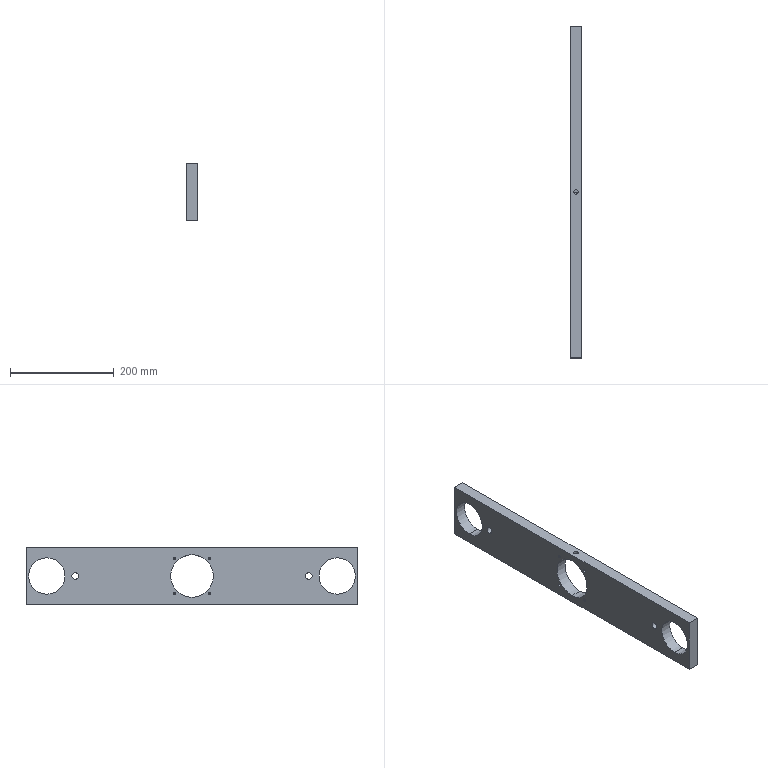Component | SolidWorks | AxisHousingBracket-2 | 1 solid | 34 faces | box 22 x 640 x 110 mm | volume 1255431 mm3 | cylinder 20 | cone 8 | plane 6 | commonest cylinder face diameters 5 x8 13 x4 70 x4 8.5 x2 82 x2
STEP:
#1=COLOUR_RGB('',0.7922,0.8196,0.9333);
#2=FILL_AREA_STYLE_COLOUR('',#1);
#3=FILL_AREA_STYLE('',(#2));
#4=SURFACE_STYLE_FILL_AREA(#3);
#5=SURFACE_SIDE_STYLE('',(#4));
#6=SURFACE_STYLE_USAGE(.BOTH.,#5);
#7=PRESENTATION_STYLE_ASSIGNMENT((#6));
#8=CARTESIAN_POINT('',(2.97,-0.1646,1.614));
#9=VERTEX_POINT('',#8);
#10=CARTESIAN_POINT('',(2.635,-0.1646,1.614));
#11=VERTEX_POINT('',#10);
#12=CARTESIAN_POINT('',(2.97,-0.1646,1.614));
#13=CARTESIAN_POINT('',(2.97,-0.1757,1.614));
#14=CARTESIAN_POINT('',(2.969,-0.1865,1.614));
#15=CARTESIAN_POINT('',(2.965,-0.2079,1.614));
#16=CARTESIAN_POINT('',(2.962,-0.2186,1.613));
#17=CARTESIAN_POINT('',(2.953,-0.2388,1.612));
#18=CARTESIAN_POINT('',(2.948,-0.2484,1.612));
#19=CARTESIAN_POINT('',(2.936,-0.2666,1.611));
#20=CARTESIAN_POINT('',(2.929,-0.2752,1.61));
#21=CARTESIAN_POINT('',(2.913,-0.2907,1.609));
#22=CARTESIAN_POINT('',(2.905,-0.2976,1.609));
#23=CARTESIAN_POINT('',(2.887,-0.3098,1.608));
#24=CARTESIAN_POINT('',(2.877,-0.315,1.607));
#25=CARTESIAN_POINT('',(2.857,-0.3233,1.606));
#26=CARTESIAN_POINT('',(2.846,-0.3266,1.606));
#27=CARTESIAN_POINT('',(2.825,-0.3309,1.606));
#28=CARTESIAN_POINT('',(2.814,-0.3319,1.605));
#29=CARTESIAN_POINT('',(2.792,-0.3319,1.605));
#30=CARTESIAN_POINT('',(2.781,-0.3308,1.606));
#31=CARTESIAN_POINT('',(2.759,-0.3266,1.606));
#32=CARTESIAN_POINT('',(2.749,-0.3234,1.606));
#33=CARTESIAN_POINT('',(2.729,-0.315,1.607));
#34=CARTESIAN_POINT('',(2.719,-0.3098,1.608));
#35=CARTESIAN_POINT('',(2.701,-0.2977,1.609));
#36=CARTESIAN_POINT('',(2.692,-0.2907,1.609));
#37=CARTESIAN_POINT('',(2.677,-0.2751,1.61));
#38=CARTESIAN_POINT('',(2.67,-0.2667,1.611));
#39=CARTESIAN_POINT('',(2.658,-0.2486,1.612));
#40=CARTESIAN_POINT('',(2.652,-0.2388,1.612));
#41=CARTESIAN_POINT('',(2.644,-0.2185,1.613));
#42=CARTESIAN_POINT('',(2.641,-0.2081,1.614));
#43=CARTESIAN_POINT('',(2.637,-0.1866,1.614));
#44=CARTESIAN_POINT('',(2.635,-0.1755,1.614));
#45=CARTESIAN_POINT('',(2.635,-0.1646,1.614));
#46=B_SPLINE_CURVE_WITH_KNOTS('',3,(#12,#13,#14,#15,#16,#17,#18,#19,#20,#21,#22,#23,#24,#25,#26,#27,#28,#29,#30,#31,#32,#33,#34,#35,#36,#37,#38,#39,#40,#41,#42,#43,#44,#45),.UNSPECIFIED.,.F.,.F.,(4,2,2,2,2,2,2,2,2,2,2,2,2,2,2,2,4),(0.,0.000831,0.001662,0.002493,0.003324,0.004155,0.004986,0.005817,0.006648,0.007479,0.00831,0.009141,0.009972,0.0108,0.01163,0.01247,0.0133),.UNSPECIFIED.);
#47=EDGE_CURVE('',#9,#11,#46,.T.);
#48=ORIENTED_EDGE('',*,*,#47,.T.);
#49=CARTESIAN_POINT('',(2.635,-0.1646,2.165));
#50=VERTEX_POINT('',#49);
#51=CARTESIAN_POINT('',(2.635,-0.1646,2.165));
#52=DIRECTION('',(0.,-0.,1.));
#53=VECTOR('',#52,39.37);
#54=LINE('',#51,#53);
#55=EDGE_CURVE('',#11,#50,#54,.T.);
#56=ORIENTED_EDGE('',*,*,#55,.T.);
#57=CARTESIAN_POINT('',(2.97,-0.1646,2.165));
#58=VERTEX_POINT('',#57);
#59=CARTESIAN_POINT('',(2.803,-0.1646,2.165));
#60=DIRECTION('',(0.,-0.,1.));
#61=DIRECTION('',(1.,0.,0.));
#62=AXIS2_PLACEMENT_3D('',#59,#60,#61);
#63=CIRCLE('',#62,0.1673);
#64=EDGE_CURVE('',#50,#58,#63,.T.);
#65=ORIENTED_EDGE('',*,*,#64,.T.);
#66=CARTESIAN_POINT('',(2.97,-0.1646,2.165));
#67=DIRECTION('',(0.,-0.,1.));
#68=VECTOR('',#67,39.37);
#69=LINE('',#66,#68);
#70=EDGE_CURVE('',#9,#58,#69,.T.);
#71=ORIENTED_EDGE('',*,*,#70,.F.);
#72=EDGE_LOOP('',(#48,#56,#65,#71));
#73=FACE_OUTER_BOUND('',#72,.T.);
#74=CARTESIAN_POINT('',(2.803,-0.1646,2.165));
#75=DIRECTION('',(0.,-0.,1.));
#76=DIRECTION('',(1.,0.,0.));
#77=AXIS2_PLACEMENT_3D('',#74,#75,#76);
#78=CYLINDRICAL_SURFACE('',#77,0.1673);
#79=ADVANCED_FACE('',(#73),#78,.F.);
#80=CARTESIAN_POINT('',(3.236,-9.023,-0.2559));
#81=VERTEX_POINT('',#80);
#82=CARTESIAN_POINT('',(3.236,-9.023,0.2559));
#83=VERTEX_POINT('',#82);
#84=CARTESIAN_POINT('',(3.236,-9.023,-0.));
#85=DIRECTION('',(-1.,0.,0.));
#86=DIRECTION('',(0.,0.,-1.));
#87=AXIS2_PLACEMENT_3D('',#84,#85,#86);
#88=CIRCLE('',#87,0.2559);
#89=EDGE_CURVE('',#81,#83,#88,.T.);
#90=ORIENTED_EDGE('',*,*,#89,.F.);
#91=CARTESIAN_POINT('',(2.37,-9.023,-0.2559));
#92=VERTEX_POINT('',#91);
#93=CARTESIAN_POINT('',(3.236,-9.023,-0.2559));
#94=DIRECTION('',(-1.,0.,0.));
#95=VECTOR('',#94,39.37);
#96=LINE('',#93,#95);
#97=EDGE_CURVE('',#81,#92,#96,.T.);
#98=ORIENTED_EDGE('',*,*,#97,.T.);
#99=CARTESIAN_POINT('',(2.37,-9.023,0.2559));
#100=VERTEX_POINT('',#99);
#101=CARTESIAN_POINT('',(2.37,-9.023,-0.));
#102=DIRECTION('',(-1.,0.,0.));
#103=DIRECTION('',(0.,0.,-1.));
#104=AXIS2_PLACEMENT_3D('',#101,#102,#103);
#105=CIRCLE('',#104,0.2559);
#106=EDGE_CURVE('',#92,#100,#105,.T.);
#107=ORIENTED_EDGE('',*,*,#106,.T.);
#108=CARTESIAN_POINT('',(3.236,-9.023,0.2559));
#109=DIRECTION('',(-1.,0.,0.));
#110=VECTOR('',#109,39.37);
#111=LINE('',#108,#110);
#112=EDGE_CURVE('',#83,#100,#111,.T.);
#113=ORIENTED_EDGE('',*,*,#112,.F.);
#114=EDGE_LOOP('',(#90,#98,#107,#113));
#115=FACE_OUTER_BOUND('',#114,.T.);
#116=CARTESIAN_POINT('',(3.236,-9.023,-0.));
#117=DIRECTION('',(-1.,0.,0.));
#118=DIRECTION('',(0.,0.,1.));
#119=AXIS2_PLACEMENT_3D('',#116,#117,#118);
#120=CYLINDRICAL_SURFACE('',#119,0.2559);
#121=ADVANCED_FACE('',(#115),#120,.F.);
#122=CARTESIAN_POINT('',(3.236,8.694,-0.2559));
#123=VERTEX_POINT('',#122);
#124=CARTESIAN_POINT('',(3.236,8.694,0.2559));
#125=VERTEX_POINT('',#124);
#126=CARTESIAN_POINT('',(3.236,8.694,0.));
#127=DIRECTION('',(-1.,0.,0.));
#128=DIRECTION('',(0.,0.,1.));
#129=AXIS2_PLACEMENT_3D('',#126,#127,#128);
#130=CIRCLE('',#129,0.2559);
#131=EDGE_CURVE('',#123,#125,#130,.T.);
#132=ORIENTED_EDGE('',*,*,#131,.F.);
#133=CARTESIAN_POINT('',(2.37,8.694,-0.2559));
#134=VERTEX_POINT('',#133);
#135=CARTESIAN_POINT('',(3.236,8.694,-0.2559));
#136=DIRECTION('',(-1.,0.,0.));
#137=VECTOR('',#136,39.37);
#138=LINE('',#135,#137);
#139=EDGE_CURVE('',#123,#134,#138,.T.);
#140=ORIENTED_EDGE('',*,*,#139,.T.);
#141=CARTESIAN_POINT('',(2.37,8.694,0.2559));
#142=VERTEX_POINT('',#141);
#143=CARTESIAN_POINT('',(2.37,8.694,0.));
#144=DIRECTION('',(-1.,0.,0.));
#145=DIRECTION('',(0.,0.,1.));
#146=AXIS2_PLACEMENT_3D('',#143,#144,#145);
#147=CIRCLE('',#146,0.2559);
#148=EDGE_CURVE('',#134,#142,#147,.T.);
#149=ORIENTED_EDGE('',*,*,#148,.T.);
#150=CARTESIAN_POINT('',(3.236,8.694,0.2559));
#151=DIRECTION('',(-1.,0.,0.));
#152=VECTOR('',#151,39.37);
#153=LINE('',#150,#152);
#154=EDGE_CURVE('',#125,#142,#153,.T.);
#155=ORIENTED_EDGE('',*,*,#154,.F.);
#156=EDGE_LOOP('',(#132,#140,#149,#155));
#157=FACE_OUTER_BOUND('',#156,.T.);
#158=CARTESIAN_POINT('',(3.236,8.694,0.));
#159=DIRECTION('',(-1.,0.,0.));
#160=DIRECTION('',(0.,0.,1.));
#161=AXIS2_PLACEMENT_3D('',#158,#159,#160);
#162=CYLINDRICAL_SURFACE('',#161,0.2559);
#163=ADVANCED_FACE('',(#157),#162,.F.);
#164=CARTESIAN_POINT('',(2.96,1.172,-1.435));
#165=VERTEX_POINT('',#164);
#166=CARTESIAN_POINT('',(2.96,1.172,-1.238));
#167=VERTEX_POINT('',#166);
#168=CARTESIAN_POINT('',(2.96,1.172,-1.336));
#169=DIRECTION('',(-1.,0.,0.));
#170=DIRECTION('',(0.,-0.,1.));
#171=AXIS2_PLACEMENT_3D('',#168,#169,#170);
#172=CIRCLE('',#171,0.09843);
#173=EDGE_CURVE('',#165,#167,#172,.T.);
#174=ORIENTED_EDGE('',*,*,#173,.F.);
#175=CARTESIAN_POINT('',(2.37,1.172,-1.435));
#176=VERTEX_POINT('',#175);
#177=CARTESIAN_POINT('',(2.37,1.172,-1.435));
#178=DIRECTION('',(-1.,0.,0.));
#179=VECTOR('',#178,39.37);
#180=LINE('',#177,#179);
#181=EDGE_CURVE('',#165,#176,#180,.T.);
#182=ORIENTED_EDGE('',*,*,#181,.T.);
#183=CARTESIAN_POINT('',(2.37,1.172,-1.238));
#184=VERTEX_POINT('',#183);
#185=CARTESIAN_POINT('',(2.37,1.172,-1.336));
#186=DIRECTION('',(-1.,0.,0.));
#187=DIRECTION('',(0.,-0.,1.));
#188=AXIS2_PLACEMENT_3D('',#185,#186,#187);
#189=CIRCLE('',#188,0.09843);
#190=EDGE_CURVE('',#176,#184,#189,.T.);
#191=ORIENTED_EDGE('',*,*,#190,.T.);
#192=CARTESIAN_POINT('',(2.37,1.172,-1.238));
#193=DIRECTION('',(-1.,0.,0.));
#194=VECTOR('',#193,39.37);
#195=LINE('',#192,#194);
#196=EDGE_CURVE('',#167,#184,#195,.T.);
#197=ORIENTED_EDGE('',*,*,#196,.F.);
#198=EDGE_LOOP('',(#174,#182,#191,#197));
#199=FACE_OUTER_BOUND('',#198,.T.);
#200=CARTESIAN_POINT('',(2.37,1.172,-1.336));
#201=DIRECTION('',(-1.,0.,0.));
#202=DIRECTION('',(0.,-0.,1.));
#203=AXIS2_PLACEMENT_3D('',#200,#201,#202);
#204=CYLINDRICAL_SURFACE('',#203,0.09843);
#205=ADVANCED_FACE('',(#199),#204,.F.);
#206=CARTESIAN_POINT('',(3.019,1.172,-1.336));
#207=VERTEX_POINT('',#206);
#208=CARTESIAN_POINT('',(2.96,1.172,-1.238));
#209=DIRECTION('',(-0.515,-0.,0.8572));
#210=VECTOR('',#209,39.37);
#211=LINE('',#208,#210);
#212=EDGE_CURVE('',#207,#167,#211,.T.);
#213=ORIENTED_EDGE('',*,*,#212,.F.);
#214=CARTESIAN_POINT('',(2.96,1.172,-1.435));
#215=DIRECTION('',(-0.515,0.,-0.8572));
#216=VECTOR('',#215,39.37);
#217=LINE('',#214,#216);
#218=EDGE_CURVE('',#207,#165,#217,.T.);
#219=ORIENTED_EDGE('',*,*,#218,.T.);
#220=ORIENTED_EDGE('',*,*,#173,.T.);
#221=EDGE_LOOP('',(#213,#219,#220));
#222=FACE_OUTER_BOUND('',#221,.T.);
#223=CARTESIAN_POINT('',(2.96,1.172,-1.336));
#224=DIRECTION('',(-1.,0.,0.));
#225=DIRECTION('',(0.,-0.,1.));
#226=AXIS2_PLACEMENT_3D('',#223,#224,#225);
#227=CONICAL_SURFACE('',#226,0.09843,1.03);
#228=ADVANCED_FACE('',(#222),#227,.F.);
#229=CARTESIAN_POINT('',(2.96,-1.501,-1.435));
#230=VERTEX_POINT('',#229);
#231=CARTESIAN_POINT('',(2.96,-1.501,-1.238));
#232=VERTEX_POINT('',#231);
#233=CARTESIAN_POINT('',(2.96,-1.501,-1.336));
#234=DIRECTION('',(-1.,0.,0.));
#235=DIRECTION('',(0.,-0.,1.));
#236=AXIS2_PLACEMENT_3D('',#233,#234,#235);
#237=CIRCLE('',#236,0.09843);
#238=EDGE_CURVE('',#230,#232,#237,.T.);
#239=ORIENTED_EDGE('',*,*,#238,.F.);
#240=CARTESIAN_POINT('',(2.37,-1.501,-1.435));
#241=VERTEX_POINT('',#240);
#242=CARTESIAN_POINT('',(2.37,-1.501,-1.435));
#243=DIRECTION('',(-1.,0.,0.));
#244=VECTOR('',#243,39.37);
#245=LINE('',#242,#244);
#246=EDGE_CURVE('',#230,#241,#245,.T.);
#247=ORIENTED_EDGE('',*,*,#246,.T.);
#248=CARTESIAN_POINT('',(2.37,-1.501,-1.238));
#249=VERTEX_POINT('',#248);
#250=CARTESIAN_POINT('',(2.37,-1.501,-1.336));
#251=DIRECTION('',(-1.,0.,0.));
#252=DIRECTION('',(0.,-0.,1.));
#253=AXIS2_PLACEMENT_3D('',#250,#251,#252);
#254=CIRCLE('',#253,0.09843);
#255=EDGE_CURVE('',#241,#249,#254,.T.);
#256=ORIENTED_EDGE('',*,*,#255,.T.);
#257=CARTESIAN_POINT('',(2.37,-1.501,-1.238));
#258=DIRECTION('',(-1.,0.,0.));
#259=VECTOR('',#258,39.37);
#260=LINE('',#257,#259);
#261=EDGE_CURVE('',#232,#249,#260,.T.);
#262=ORIENTED_EDGE('',*,*,#261,.F.);
#263=EDGE_LOOP('',(#239,#247,#256,#262));
#264=FACE_OUTER_BOUND('',#263,.T.);
#265=CARTESIAN_POINT('',(2.37,-1.501,-1.336));
#266=DIRECTION('',(-1.,0.,0.));
#267=DIRECTION('',(0.,-0.,1.));
#268=AXIS2_PLACEMENT_3D('',#265,#266,#267);
#269=CYLINDRICAL_SURFACE('',#268,0.09843);
#270=ADVANCED_FACE('',(#264),#269,.F.);
#271=CARTESIAN_POINT('',(3.019,-1.501,-1.336));
#272=VERTEX_POINT('',#271);
#273=CARTESIAN_POINT('',(2.96,-1.501,-1.238));
#274=DIRECTION('',(-0.515,-0.,0.8572));
#275=VECTOR('',#274,39.37);
#276=LINE('',#273,#275);
#277=EDGE_CURVE('',#272,#232,#276,.T.);
#278=ORIENTED_EDGE('',*,*,#277,.F.);
#279=CARTESIAN_POINT('',(2.96,-1.501,-1.435));
#280=DIRECTION('',(-0.515,0.,-0.8572));
#281=VECTOR('',#280,39.37);
#282=LINE('',#279,#281);
#283=EDGE_CURVE('',#272,#230,#282,.T.);
#284=ORIENTED_EDGE('',*,*,#283,.T.);
#285=ORIENTED_EDGE('',*,*,#238,.T.);
#286=EDGE_LOOP('',(#278,#284,#285));
#287=FACE_OUTER_BOUND('',#286,.T.);
#288=CARTESIAN_POINT('',(2.96,-1.501,-1.336));
#289=DIRECTION('',(-1.,0.,0.));
#290=DIRECTION('',(0.,-0.,1.));
#291=AXIS2_PLACEMENT_3D('',#288,#289,#290);
#292=CONICAL_SURFACE('',#291,0.09843,1.03);
#293=ADVANCED_FACE('',(#287),#292,.F.);
#294=CARTESIAN_POINT('',(2.96,-1.501,1.238));
#295=VERTEX_POINT('',#294);
#296=CARTESIAN_POINT('',(2.96,-1.501,1.435));
#297=VERTEX_POINT('',#296);
#298=CARTESIAN_POINT('',(2.96,-1.501,1.336));
#299=DIRECTION('',(-1.,0.,0.));
#300=DIRECTION('',(0.,-0.,1.));
#301=AXIS2_PLACEMENT_3D('',#298,#299,#300);
#302=CIRCLE('',#301,0.09843);
#303=EDGE_CURVE('',#295,#297,#302,.T.);
#304=ORIENTED_EDGE('',*,*,#303,.F.);
#305=CARTESIAN_POINT('',(2.37,-1.501,1.238));
#306=VERTEX_POINT('',#305);
#307=CARTESIAN_POINT('',(2.37,-1.501,1.238));
#308=DIRECTION('',(-1.,0.,0.));
#309=VECTOR('',#308,39.37);
#310=LINE('',#307,#309);
#311=EDGE_CURVE('',#295,#306,#310,.T.);
#312=ORIENTED_EDGE('',*,*,#311,.T.);
#313=CARTESIAN_POINT('',(2.37,-1.501,1.435));
#314=VERTEX_POINT('',#313);
#315=CARTESIAN_POINT('',(2.37,-1.501,1.336));
#316=DIRECTION('',(-1.,0.,0.));
#317=DIRECTION('',(0.,-0.,1.));
#318=AXIS2_PLACEMENT_3D('',#315,#316,#317);
#319=CIRCLE('',#318,0.09843);
#320=EDGE_CURVE('',#306,#314,#319,.T.);
#321=ORIENTED_EDGE('',*,*,#320,.T.);
#322=CARTESIAN_POINT('',(2.37,-1.501,1.435));
#323=DIRECTION('',(-1.,0.,0.));
#324=VECTOR('',#323,39.37);
#325=LINE('',#322,#324);
#326=EDGE_CURVE('',#297,#314,#325,.T.);
#327=ORIENTED_EDGE('',*,*,#326,.F.);
#328=EDGE_LOOP('',(#304,#312,#321,#327));
#329=FACE_OUTER_BOUND('',#328,.T.);
#330=CARTESIAN_POINT('',(2.37,-1.501,1.336));
#331=DIRECTION('',(-1.,0.,0.));
#332=DIRECTION('',(0.,-0.,1.));
#333=AXIS2_PLACEMENT_3D('',#330,#331,#332);
#334=CYLINDRICAL_SURFACE('',#333,0.09843);
#335=ADVANCED_FACE('',(#329),#334,.F.);
#336=CARTESIAN_POINT('',(3.019,-1.501,1.336));
#337=VERTEX_POINT('',#336);
#338=CARTESIAN_POINT('',(2.96,-1.501,1.435));
#339=DIRECTION('',(-0.515,-0.,0.8572));
#340=VECTOR('',#339,39.37);
#341=LINE('',#338,#340);
#342=EDGE_CURVE('',#337,#297,#341,.T.);
#343=ORIENTED_EDGE('',*,*,#342,.F.);
#344=CARTESIAN_POINT('',(2.96,-1.501,1.238));
#345=DIRECTION('',(-0.515,0.,-0.8572));
#346=VECTOR('',#345,39.37);
#347=LINE('',#344,#346);
#348=EDGE_CURVE('',#337,#295,#347,.T.);
#349=ORIENTED_EDGE('',*,*,#348,.T.);
#350=ORIENTED_EDGE('',*,*,#303,.T.);
#351=EDGE_LOOP('',(#343,#349,#350));
#352=FACE_OUTER_BOUND('',#351,.T.);
#353=CARTESIAN_POINT('',(2.96,-1.501,1.336));
#354=DIRECTION('',(-1.,0.,0.));
#355=DIRECTION('',(0.,-0.,1.));
#356=AXIS2_PLACEMENT_3D('',#353,#354,#355);
#357=CONICAL_SURFACE('',#356,0.09843,1.03);
#358=ADVANCED_FACE('',(#352),#357,.F.);
#359=CARTESIAN_POINT('',(2.96,1.172,1.238));
#360=VERTEX_POINT('',#359);
#361=CARTESIAN_POINT('',(2.96,1.172,1.435));
#362=VERTEX_POINT('',#361);
#363=CARTESIAN_POINT('',(2.96,1.172,1.336));
#364=DIRECTION('',(-1.,0.,0.));
#365=DIRECTION('',(0.,-0.,1.));
#366=AXIS2_PLACEMENT_3D('',#363,#364,#365);
#367=CIRCLE('',#366,0.09843);
#368=EDGE_CURVE('',#360,#362,#367,.T.);
#369=ORIENTED_EDGE('',*,*,#368,.F.);
#370=CARTESIAN_POINT('',(2.37,1.172,1.238));
#371=VERTEX_POINT('',#370);
#372=CARTESIAN_POINT('',(2.37,1.172,1.238));
#373=DIRECTION('',(-1.,0.,0.));
#374=VECTOR('',#373,39.37);
#375=LINE('',#372,#374);
#376=EDGE_CURVE('',#360,#371,#375,.T.);
#377=ORIENTED_EDGE('',*,*,#376,.T.);
#378=CARTESIAN_POINT('',(2.37,1.172,1.435));
#379=VERTEX_POINT('',#378);
#380=CARTESIAN_POINT('',(2.37,1.172,1.336));
#381=DIRECTION('',(-1.,0.,0.));
#382=DIRECTION('',(0.,-0.,1.));
#383=AXIS2_PLACEMENT_3D('',#380,#381,#382);
#384=CIRCLE('',#383,0.09843);
#385=EDGE_CURVE('',#371,#379,#384,.T.);
#386=ORIENTED_EDGE('',*,*,#385,.T.);
#387=CARTESIAN_POINT('',(2.37,1.172,1.435));
#388=DIRECTION('',(-1.,0.,0.));
#389=VECTOR('',#388,39.37);
#390=LINE('',#387,#389);
#391=EDGE_CURVE('',#362,#379,#390,.T.);
#392=ORIENTED_EDGE('',*,*,#391,.F.);
#393=EDGE_LOOP('',(#369,#377,#386,#392));
#394=FACE_OUTER_BOUND('',#393,.T.);
#395=CARTESIAN_POINT('',(2.37,1.172,1.336));
#396=DIRECTION('',(-1.,0.,0.));
#397=DIRECTION('',(0.,-0.,1.));
#398=AXIS2_PLACEMENT_3D('',#395,#396,#397);
#399=CYLINDRICAL_SURFACE('',#398,0.09843);
#400=ADVANCED_FACE('',(#394),#399,.F.);
#401=CARTESIAN_POINT('',(3.019,1.172,1.336));
#402=VERTEX_POINT('',#401);
#403=CARTESIAN_POINT('',(2.96,1.172,1.435));
#404=DIRECTION('',(-0.515,-0.,0.8572));
#405=VECTOR('',#404,39.37);
#406=LINE('',#403,#405);
#407=EDGE_CURVE('',#402,#362,#406,.T.);
#408=ORIENTED_EDGE('',*,*,#407,.F.);
#409=CARTESIAN_POINT('',(2.96,1.172,1.238));
#410=DIRECTION('',(-0.515,0.,-0.8572));
#411=VECTOR('',#410,39.37);
#412=LINE('',#409,#411);
#413=EDGE_CURVE('',#402,#360,#412,.T.);
#414=ORIENTED_EDGE('',*,*,#413,.T.);
#415=ORIENTED_EDGE('',*,*,#368,.T.);
#416=EDGE_LOOP('',(#408,#414,#415));
#417=FACE_OUTER_BOUND('',#416,.T.);
#418=CARTESIAN_POINT('',(2.96,1.172,1.336));
#419=DIRECTION('',(-1.,0.,0.));
#420=DIRECTION('',(0.,-0.,1.));
#421=AXIS2_PLACEMENT_3D('',#418,#419,#420);
#422=CONICAL_SURFACE('',#421,0.09843,1.03);
#423=ADVANCED_FACE('',(#417),#422,.F.);
#424=CARTESIAN_POINT('',(2.37,-11.188,-1.378));
#425=VERTEX_POINT('',#424);
#426=CARTESIAN_POINT('',(2.37,-11.188,1.378));
#427=VERTEX_POINT('',#426);
#428=CARTESIAN_POINT('',(2.37,-11.188,-0.));
#429=DIRECTION('',(-1.,0.,0.));
#430=DIRECTION('',(0.,0.,-1.));
#431=AXIS2_PLACEMENT_3D('',#428,#429,#430);
#432=CIRCLE('',#431,1.378);
#433=EDGE_CURVE('',#425,#427,#432,.T.);
#434=ORIENTED_EDGE('',*,*,#433,.T.);
#435=CARTESIAN_POINT('',(3.236,-11.188,1.378));
#436=VERTEX_POINT('',#435);
#437=CARTESIAN_POINT('',(2.37,-11.188,1.378));
#438=DIRECTION('',(1.,0.,0.));
#439=VECTOR('',#438,39.37);
#440=LINE('',#437,#439);
#441=EDGE_CURVE('',#427,#436,#440,.T.);
#442=ORIENTED_EDGE('',*,*,#441,.T.);
#443=CARTESIAN_POINT('',(3.236,-11.188,-1.378));
#444=VERTEX_POINT('',#443);
#445=CARTESIAN_POINT('',(3.236,-11.188,-0.));
#446=DIRECTION('',(-1.,0.,0.));
#447=DIRECTION('',(0.,0.,-1.));
#448=AXIS2_PLACEMENT_3D('',#445,#446,#447);
#449=CIRCLE('',#448,1.378);
#450=EDGE_CURVE('',#444,#436,#449,.T.);
#451=ORIENTED_EDGE('',*,*,#450,.F.);
#452=CARTESIAN_POINT('',(2.37,-11.188,-1.378));
#453=DIRECTION('',(1.,0.,0.));
#454=VECTOR('',#453,39.37);
#455=LINE('',#452,#454);
#456=EDGE_CURVE('',#425,#444,#455,.T.);
#457=ORIENTED_EDGE('',*,*,#456,.F.);
#458=EDGE_LOOP('',(#434,#442,#451,#457));
#459=FACE_OUTER_BOUND('',#458,.T.);
#460=CARTESIAN_POINT('',(2.37,-11.188,-0.));
#461=DIRECTION('',(1.,0.,0.));
#462=DIRECTION('',(0.,0.,-1.));
#463=AXIS2_PLACEMENT_3D('',#460,#461,#462);
#464=CYLINDRICAL_SURFACE('',#463,1.378);
#465=ADVANCED_FACE('',(#459),#464,.F.);
#466=CARTESIAN_POINT('',(2.37,10.859,-1.378));
#467=VERTEX_POINT('',#466);
#468=CARTESIAN_POINT('',(2.37,10.859,1.378));
#469=VERTEX_POINT('',#468);
#470=CARTESIAN_POINT('',(2.37,10.859,0.));
#471=DIRECTION('',(-1.,0.,0.));
#472=DIRECTION('',(0.,-0.,1.));
#473=AXIS2_PLACEMENT_3D('',#470,#471,#472);
#474=CIRCLE('',#473,1.378);
#475=EDGE_CURVE('',#467,#469,#474,.T.);
#476=ORIENTED_EDGE('',*,*,#475,.T.);
#477=CARTESIAN_POINT('',(3.236,10.859,1.378));
#478=VERTEX_POINT('',#477);
#479=CARTESIAN_POINT('',(2.37,10.859,1.378));
#480=DIRECTION('',(1.,0.,0.));
#481=VECTOR('',#480,39.37);
#482=LINE('',#479,#481);
#483=EDGE_CURVE('',#469,#478,#482,.T.);
#484=ORIENTED_EDGE('',*,*,#483,.T.);
#485=CARTESIAN_POINT('',(3.236,10.859,-1.378));
#486=VERTEX_POINT('',#485);
#487=CARTESIAN_POINT('',(3.236,10.859,0.));
#488=DIRECTION('',(-1.,0.,0.));
#489=DIRECTION('',(0.,-0.,1.));
#490=AXIS2_PLACEMENT_3D('',#487,#488,#489);
#491=CIRCLE('',#490,1.378);
#492=EDGE_CURVE('',#486,#478,#491,.T.);
#493=ORIENTED_EDGE('',*,*,#492,.F.);
#494=CARTESIAN_POINT('',(2.37,10.859,-1.378));
#495=DIRECTION('',(1.,0.,0.));
#496=VECTOR('',#495,39.37);
#497=LINE('',#494,#496);
#498=EDGE_CURVE('',#467,#486,#497,.T.);
#499=ORIENTED_EDGE('',*,*,#498,.F.);
#500=EDGE_LOOP('',(#476,#484,#493,#499));
#501=FACE_OUTER_BOUND('',#500,.T.);
#502=CARTESIAN_POINT('',(2.37,10.859,0.));
#503=DIRECTION('',(1.,0.,0.));
#504=DIRECTION('',(0.,0.,-1.));
#505=AXIS2_PLACEMENT_3D('',#502,#503,#504);
#506=CYLINDRICAL_SURFACE('',#505,1.378);
#507=ADVANCED_FACE('',(#501),#506,.F.);
#508=CARTESIAN_POINT('',(2.37,-0.1646,-1.614));
#509=VERTEX_POINT('',#508);
#510=CARTESIAN_POINT('',(2.37,-0.1646,1.614));
#511=VERTEX_POINT('',#510);
#512=CARTESIAN_POINT('',(2.37,-0.1646,0.));
#513=DIRECTION('',(-1.,0.,0.));
#514=DIRECTION('',(0.,-0.,1.));
#515=AXIS2_PLACEMENT_3D('',#512,#513,#514);
#516=CIRCLE('',#515,1.614);
#517=EDGE_CURVE('',#509,#511,#516,.T.);
#518=ORIENTED_EDGE('',*,*,#517,.T.);
#519=CARTESIAN_POINT('',(2.37,-0.1646,1.614));
#520=DIRECTION('',(1.,0.,0.));
#521=VECTOR('',#520,39.37);
#522=LINE('',#519,#521);
#523=EDGE_CURVE('',#511,#11,#522,.T.);
#524=ORIENTED_EDGE('',*,*,#523,.T.);
#525=ORIENTED_EDGE('',*,*,#47,.F.);
#526=CARTESIAN_POINT('',(3.236,-0.1646,1.614));
#527=VERTEX_POINT('',#526);
#528=CARTESIAN_POINT('',(2.37,-0.1646,1.614));
#529=DIRECTION('',(1.,0.,0.));
#530=VECTOR('',#529,39.37);
#531=LINE('',#528,#530);
#532=EDGE_CURVE('',#9,#527,#531,.T.);
#533=ORIENTED_EDGE('',*,*,#532,.T.);
#534=CARTESIAN_POINT('',(3.236,-0.1646,-1.614));
#535=VERTEX_POINT('',#534);
#536=CARTESIAN_POINT('',(3.236,-0.1646,0.));
#537=DIRECTION('',(-1.,0.,0.));
#538=DIRECTION('',(0.,-0.,1.));
#539=AXIS2_PLACEMENT_3D('',#536,#537,#538);
#540=CIRCLE('',#539,1.614);
#541=EDGE_CURVE('',#535,#527,#540,.T.);
#542=ORIENTED_EDGE('',*,*,#541,.F.);
#543=CARTESIAN_POINT('',(2.37,-0.1646,-1.614));
#544=DIRECTION('',(1.,0.,0.));
#545=VECTOR('',#544,39.37);
#546=LINE('',#543,#545);
#547=EDGE_CURVE('',#509,#535,#546,.T.);
#548=ORIENTED_EDGE('',*,*,#547,.F.);
#549=EDGE_LOOP('',(#518,#524,#525,#533,#542,#548));
#550=FACE_OUTER_BOUND('',#549,.T.);
#551=CARTESIAN_POINT('',(2.37,-0.1646,0.));
#552=DIRECTION('',(1.,0.,0.));
#553=DIRECTION('',(0.,0.,-1.));
#554=AXIS2_PLACEMENT_3D('',#551,#552,#553);
#555=CYLINDRICAL_SURFACE('',#554,1.614);
#556=ADVANCED_FACE('',(#550),#555,.F.);
#557=CARTESIAN_POINT('',(2.37,-9.023,-0.));
#558=DIRECTION('',(-1.,0.,0.));
#559=DIRECTION('',(0.,0.,-1.));
#560=AXIS2_PLACEMENT_3D('',#557,#558,#559);
#561=CIRCLE('',#560,0.2559);
#562=EDGE_CURVE('',#100,#92,#561,.T.);
#563=ORIENTED_EDGE('',*,*,#562,.F.);
#564=ORIENTED_EDGE('',*,*,#106,.F.);
#565=EDGE_LOOP('',(#563,#564));
#566=FACE_BOUND('',#565,.T.);
#567=CARTESIAN_POINT('',(2.37,8.694,0.));
#568=DIRECTION('',(-1.,0.,0.));
#569=DIRECTION('',(0.,0.,1.));
#570=AXIS2_PLACEMENT_3D('',#567,#568,#569);
#571=CIRCLE('',#570,0.2559);
#572=EDGE_CURVE('',#142,#134,#571,.T.);
#573=ORIENTED_EDGE('',*,*,#572,.F.);
#574=ORIENTED_EDGE('',*,*,#148,.F.);
#575=EDGE_LOOP('',(#573,#574));
#576=FACE_BOUND('',#575,.T.);
#577=CARTESIAN_POINT('',(2.37,1.172,-1.336));
#578=DIRECTION('',(-1.,0.,0.));
#579=DIRECTION('',(0.,-0.,1.));
#580=AXIS2_PLACEMENT_3D('',#577,#578,#579);
#581=CIRCLE('',#580,0.09843);
#582=EDGE_CURVE('',#184,#176,#581,.T.);
#583=ORIENTED_EDGE('',*,*,#582,.F.);
#584=ORIENTED_EDGE('',*,*,#190,.F.);
#585=EDGE_LOOP('',(#583,#584));
#586=FACE_BOUND('',#585,.T.);
#587=CARTESIAN_POINT('',(2.37,-1.501,-1.336));
#588=DIRECTION('',(-1.,0.,0.));
#589=DIRECTION('',(0.,-0.,1.));
#590=AXIS2_PLACEMENT_3D('',#587,#588,#589);
#591=CIRCLE('',#590,0.09843);
#592=EDGE_CURVE('',#249,#241,#591,.T.);
#593=ORIENTED_EDGE('',*,*,#592,.F.);
#594=ORIENTED_EDGE('',*,*,#255,.F.);
#595=EDGE_LOOP('',(#593,#594));
#596=FACE_BOUND('',#595,.T.);
#597=CARTESIAN_POINT('',(2.37,-1.501,1.336));
#598=DIRECTION('',(-1.,0.,0.));
#599=DIRECTION('',(0.,-0.,1.));
#600=AXIS2_PLACEMENT_3D('',#597,#598,#599);
#601=CIRCLE('',#600,0.09843);
#602=EDGE_CURVE('',#314,#306,#601,.T.);
#603=ORIENTED_EDGE('',*,*,#602,.F.);
#604=ORIENTED_EDGE('',*,*,#320,.F.);
#605=EDGE_LOOP('',(#603,#604));
#606=FACE_BOUND('',#605,.T.);
#607=CARTESIAN_POINT('',(2.37,1.172,1.336));
#608=DIRECTION('',(-1.,0.,0.));
#609=DIRECTION('',(0.,-0.,1.));
#610=AXIS2_PLACEMENT_3D('',#607,#608,#609);
#611=CIRCLE('',#610,0.09843);
#612=EDGE_CURVE('',#379,#371,#611,.T.);
#613=ORIENTED_EDGE('',*,*,#612,.F.);
#614=ORIENTED_EDGE('',*,*,#385,.F.);
#615=EDGE_LOOP('',(#613,#614));
#616=FACE_BOUND('',#615,.T.);
#617=ORIENTED_EDGE('',*,*,#475,.F.);
#618=CARTESIAN_POINT('',(2.37,10.859,0.));
#619=DIRECTION('',(-1.,0.,0.));
#620=DIRECTION('',(0.,-0.,1.));
#621=AXIS2_PLACEMENT_3D('',#618,#619,#620);
#622=CIRCLE('',#621,1.378);
#623=EDGE_CURVE('',#469,#467,#622,.T.);
#624=ORIENTED_EDGE('',*,*,#623,.F.);
#625=EDGE_LOOP('',(#617,#624));
#626=FACE_BOUND('',#625,.T.);
#627=CARTESIAN_POINT('',(2.37,-12.763,2.165));
#628=VERTEX_POINT('',#627);
#629=CARTESIAN_POINT('',(2.37,12.434,2.165));
#630=VERTEX_POINT('',#629);
#631=CARTESIAN_POINT('',(2.37,12.434,2.165));
#632=DIRECTION('',(0.,1.,0.));
#633=VECTOR('',#632,39.37);
#634=LINE('',#631,#633);
#635=EDGE_CURVE('',#628,#630,#634,.T.);
#636=ORIENTED_EDGE('',*,*,#635,.T.);
#637=CARTESIAN_POINT('',(2.37,12.434,-2.165));
#638=VERTEX_POINT('',#637);
#639=CARTESIAN_POINT('',(2.37,12.434,-2.165));
#640=DIRECTION('',(0.,0.,-1.));
#641=VECTOR('',#640,39.37);
#642=LINE('',#639,#641);
#643=EDGE_CURVE('',#630,#638,#642,.T.);
#644=ORIENTED_EDGE('',*,*,#643,.T.);
#645=CARTESIAN_POINT('',(2.37,-12.763,-2.165));
#646=VERTEX_POINT('',#645);
#647=CARTESIAN_POINT('',(2.37,12.434,-2.165));
#648=DIRECTION('',(0.,-1.,-0.));
#649=VECTOR('',#648,39.37);
#650=LINE('',#647,#649);
#651=EDGE_CURVE('',#638,#646,#650,.T.);
#652=ORIENTED_EDGE('',*,*,#651,.T.);
#653=CARTESIAN_POINT('',(2.37,-12.763,-2.165));
#654=DIRECTION('',(0.,-0.,1.));
#655=VECTOR('',#654,39.37);
#656=LINE('',#653,#655);
#657=EDGE_CURVE('',#646,#628,#656,.T.);
#658=ORIENTED_EDGE('',*,*,#657,.T.);
#659=EDGE_LOOP('',(#636,#644,#652,#658));
#660=FACE_OUTER_BOUND('',#659,.T.);
#661=ORIENTED_EDGE('',*,*,#517,.F.);
#662=CARTESIAN_POINT('',(2.37,-0.1646,0.));
#663=DIRECTION('',(-1.,0.,0.));
#664=DIRECTION('',(0.,-0.,1.));
#665=AXIS2_PLACEMENT_3D('',#662,#663,#664);
#666=CIRCLE('',#665,1.614);
#667=EDGE_CURVE('',#511,#509,#666,.T.);
#668=ORIENTED_EDGE('',*,*,#667,.F.);
#669=EDGE_LOOP('',(#661,#668));
#670=FACE_BOUND('',#669,.T.);
#671=ORIENTED_EDGE('',*,*,#433,.F.);
#672=CARTESIAN_POINT('',(2.37,-11.188,-0.));
#673=DIRECTION('',(-1.,0.,0.));
#674=DIRECTION('',(0.,0.,-1.));
#675=AXIS2_PLACEMENT_3D('',#672,#673,#674);
#676=CIRCLE('',#675,1.378);
#677=EDGE_CURVE('',#427,#425,#676,.T.);
#678=ORIENTED_EDGE('',*,*,#677,.F.);
#679=EDGE_LOOP('',(#671,#678));
#680=FACE_BOUND('',#679,.T.);
#681=CARTESIAN_POINT('',(2.37,-12.763,2.165));
#682=DIRECTION('',(-1.,0.,0.));
#683=DIRECTION('',(0.,-0.,1.));
#684=AXIS2_PLACEMENT_3D('',#681,#682,#683);
#685=PLANE('',#684);
#686=ADVANCED_FACE('',(#566,#576,#586,#596,#606,#616,#626,#660,#670,#680),#685,.T.);
#687=CARTESIAN_POINT('',(3.236,-9.023,-0.));
#688=DIRECTION('',(-1.,0.,0.));
#689=DIRECTION('',(0.,0.,-1.));
#690=AXIS2_PLACEMENT_3D('',#687,#688,#689);
#691=CIRCLE('',#690,0.2559);
#692=EDGE_CURVE('',#83,#81,#691,.T.);
#693=ORIENTED_EDGE('',*,*,#692,.T.);
#694=ORIENTED_EDGE('',*,*,#89,.T.);
#695=EDGE_LOOP('',(#693,#694));
#696=FACE_BOUND('',#695,.T.);
#697=CARTESIAN_POINT('',(3.236,8.694,0.));
#698=DIRECTION('',(-1.,0.,0.));
#699=DIRECTION('',(0.,0.,1.));
#700=AXIS2_PLACEMENT_3D('',#697,#698,#699);
#701=CIRCLE('',#700,0.2559);
#702=EDGE_CURVE('',#125,#123,#701,.T.);
#703=ORIENTED_EDGE('',*,*,#702,.T.);
#704=ORIENTED_EDGE('',*,*,#131,.T.);
#705=EDGE_LOOP('',(#703,#704));
#706=FACE_BOUND('',#705,.T.);
#707=CARTESIAN_POINT('',(3.236,-12.763,2.165));
#708=VERTEX_POINT('',#707);
#709=CARTESIAN_POINT('',(3.236,12.434,2.165));
#710=VERTEX_POINT('',#709);
#711=CARTESIAN_POINT('',(3.236,12.434,2.165));
#712=DIRECTION('',(0.,1.,0.));
#713=VECTOR('',#712,39.37);
#714=LINE('',#711,#713);
#715=EDGE_CURVE('',#708,#710,#714,.T.);
#716=ORIENTED_EDGE('',*,*,#715,.F.);
#717=CARTESIAN_POINT('',(3.236,-12.763,-2.165));
#718=VERTEX_POINT('',#717);
#719=CARTESIAN_POINT('',(3.236,-12.763,-2.165));
#720=DIRECTION('',(0.,-0.,1.));
#721=VECTOR('',#720,39.37);
#722=LINE('',#719,#721);
#723=EDGE_CURVE('',#718,#708,#722,.T.);
#724=ORIENTED_EDGE('',*,*,#723,.F.);
#725=CARTESIAN_POINT('',(3.236,12.434,-2.165));
#726=VERTEX_POINT('',#725);
#727=CARTESIAN_POINT('',(3.236,12.434,-2.165));
#728=DIRECTION('',(0.,-1.,-0.));
#729=VECTOR('',#728,39.37);
#730=LINE('',#727,#729);
#731=EDGE_CURVE('',#726,#718,#730,.T.);
#732=ORIENTED_EDGE('',*,*,#731,.F.);
#733=CARTESIAN_POINT('',(3.236,12.434,-2.165));
#734=DIRECTION('',(0.,0.,-1.));
#735=VECTOR('',#734,39.37);
#736=LINE('',#733,#735);
#737=EDGE_CURVE('',#710,#726,#736,.T.);
#738=ORIENTED_EDGE('',*,*,#737,.F.);
#739=EDGE_LOOP('',(#716,#724,#732,#738));
#740=FACE_OUTER_BOUND('',#739,.T.);
#741=ORIENTED_EDGE('',*,*,#541,.T.);
#742=CARTESIAN_POINT('',(3.236,-0.1646,0.));
#743=DIRECTION('',(-1.,0.,0.));
#744=DIRECTION('',(0.,-0.,1.));
#745=AXIS2_PLACEMENT_3D('',#742,#743,#744);
#746=CIRCLE('',#745,1.614);
#747=EDGE_CURVE('',#527,#535,#746,.T.);
#748=ORIENTED_EDGE('',*,*,#747,.T.);
#749=EDGE_LOOP('',(#741,#748));
#750=FACE_BOUND('',#749,.T.);
#751=ORIENTED_EDGE('',*,*,#492,.T.);
#752=CARTESIAN_POINT('',(3.236,10.859,0.));
#753=DIRECTION('',(-1.,0.,0.));
#754=DIRECTION('',(0.,-0.,1.));
#755=AXIS2_PLACEMENT_3D('',#752,#753,#754);
#756=CIRCLE('',#755,1.378);
#757=EDGE_CURVE('',#478,#486,#756,.T.);
#758=ORIENTED_EDGE('',*,*,#757,.T.);
#759=EDGE_LOOP('',(#751,#758));
#760=FACE_BOUND('',#759,.T.);
#761=ORIENTED_EDGE('',*,*,#450,.T.);
#762=CARTESIAN_POINT('',(3.236,-11.188,-0.));
#763=DIRECTION('',(-1.,0.,0.));
#764=DIRECTION('',(0.,0.,-1.));
#765=AXIS2_PLACEMENT_3D('',#762,#763,#764);
#766=CIRCLE('',#765,1.378);
#767=EDGE_CURVE('',#436,#444,#766,.T.);
#768=ORIENTED_EDGE('',*,*,#767,.T.);
#769=EDGE_LOOP('',(#761,#768));
#770=FACE_BOUND('',#769,.T.);
#771=CARTESIAN_POINT('',(3.236,-12.763,2.165));
#772=DIRECTION('',(-1.,0.,0.));
#773=DIRECTION('',(0.,-0.,1.));
#774=AXIS2_PLACEMENT_3D('',#771,#772,#773);
#775=PLANE('',#774);
#776=ADVANCED_FACE('',(#696,#706,#740,#750,#760,#770),#775,.F.);
#777=CARTESIAN_POINT('',(2.803,-0.1646,2.165));
#778=DIRECTION('',(0.,-0.,1.));
#779=DIRECTION('',(1.,0.,0.));
#780=AXIS2_PLACEMENT_3D('',#777,#778,#779);
#781=CIRCLE('',#780,0.1673);
#782=EDGE_CURVE('',#58,#50,#781,.T.);
#783=ORIENTED_EDGE('',*,*,#782,.F.);
#784=ORIENTED_EDGE('',*,*,#64,.F.);
#785=EDGE_LOOP('',(#783,#784));
#786=FACE_BOUND('',#785,.T.);
#787=ORIENTED_EDGE('',*,*,#715,.T.);
#788=CARTESIAN_POINT('',(2.37,12.434,2.165));
#789=DIRECTION('',(1.,0.,0.));
#790=VECTOR('',#789,39.37);
#791=LINE('',#788,#790);
#792=EDGE_CURVE('',#630,#710,#791,.T.);
#793=ORIENTED_EDGE('',*,*,#792,.F.);
#794=ORIENTED_EDGE('',*,*,#635,.F.);
#795=CARTESIAN_POINT('',(2.37,-12.763,2.165));
#796=DIRECTION('',(1.,0.,0.));
#797=VECTOR('',#796,39.37);
#798=LINE('',#795,#797);
#799=EDGE_CURVE('',#628,#708,#798,.T.);
#800=ORIENTED_EDGE('',*,*,#799,.T.);
#801=EDGE_LOOP('',(#787,#793,#794,#800));
#802=FACE_OUTER_BOUND('',#801,.T.);
#803=CARTESIAN_POINT('',(2.37,12.434,2.165));
#804=DIRECTION('',(0.,0.,-1.));
#805=DIRECTION('',(0.,-1.,-0.));
#806=AXIS2_PLACEMENT_3D('',#803,#804,#805);
#807=PLANE('',#806);
#808=ADVANCED_FACE('',(#786,#802),#807,.F.);
#809=ORIENTED_EDGE('',*,*,#737,.T.);
#810=CARTESIAN_POINT('',(2.37,12.434,-2.165));
#811=DIRECTION('',(1.,0.,0.));
#812=VECTOR('',#811,39.37);
#813=LINE('',#810,#812);
#814=EDGE_CURVE('',#638,#726,#813,.T.);
#815=ORIENTED_EDGE('',*,*,#814,.F.);
#816=ORIENTED_EDGE('',*,*,#643,.F.);
#817=ORIENTED_EDGE('',*,*,#792,.T.);
#818=EDGE_LOOP('',(#809,#815,#816,#817));
#819=FACE_OUTER_BOUND('',#818,.T.);
#820=CARTESIAN_POINT('',(2.37,12.434,-2.165));
#821=DIRECTION('',(0.,-1.,-0.));
#822=DIRECTION('',(1.,0.,0.));
#823=AXIS2_PLACEMENT_3D('',#820,#821,#822);
#824=PLANE('',#823);
#825=ADVANCED_FACE('',(#819),#824,.F.);
#826=ORIENTED_EDGE('',*,*,#731,.T.);
#827=CARTESIAN_POINT('',(2.37,-12.763,-2.165));
#828=DIRECTION('',(1.,0.,0.));
#829=VECTOR('',#828,39.37);
#830=LINE('',#827,#829);
#831=EDGE_CURVE('',#646,#718,#830,.T.);
#832=ORIENTED_EDGE('',*,*,#831,.F.);
#833=ORIENTED_EDGE('',*,*,#651,.F.);
#834=ORIENTED_EDGE('',*,*,#814,.T.);
#835=EDGE_LOOP('',(#826,#832,#833,#834));
#836=FACE_OUTER_BOUND('',#835,.T.);
#837=CARTESIAN_POINT('',(2.37,12.434,-2.165));
#838=DIRECTION('',(0.,-0.,1.));
#839=DIRECTION('',(0.,1.,0.));
#840=AXIS2_PLACEMENT_3D('',#837,#838,#839);
#841=PLANE('',#840);
#842=ADVANCED_FACE('',(#836),#841,.F.);
#843=ORIENTED_EDGE('',*,*,#723,.T.);
#844=ORIENTED_EDGE('',*,*,#799,.F.);
#845=ORIENTED_EDGE('',*,*,#657,.F.);
#846=ORIENTED_EDGE('',*,*,#831,.T.);
#847=EDGE_LOOP('',(#843,#844,#845,#846));
#848=FACE_OUTER_BOUND('',#847,.T.);
#849=CARTESIAN_POINT('',(2.37,-12.763,-2.165));
#850=DIRECTION('',(0.,1.,0.));
#851=DIRECTION('',(-1.,0.,0.));
#852=AXIS2_PLACEMENT_3D('',#849,#850,#851);
#853=PLANE('',#852);
#854=ADVANCED_FACE('',(#848),#853,.F.);
#855=ORIENTED_EDGE('',*,*,#523,.F.);
#856=ORIENTED_EDGE('',*,*,#667,.T.);
#857=ORIENTED_EDGE('',*,*,#547,.T.);
#858=ORIENTED_EDGE('',*,*,#747,.F.);
#859=ORIENTED_EDGE('',*,*,#532,.F.);
#860=CARTESIAN_POINT('',(2.635,-0.1646,1.614));
#861=CARTESIAN_POINT('',(2.635,-0.1537,1.614));
#862=CARTESIAN_POINT('',(2.637,-0.1428,1.614));
#863=CARTESIAN_POINT('',(2.641,-0.1212,1.614));
#864=CARTESIAN_POINT('',(2.644,-0.1107,1.613));
#865=CARTESIAN_POINT('',(2.652,-0.09053,1.613));
#866=CARTESIAN_POINT('',(2.658,-0.0808,1.612));
#867=CARTESIAN_POINT('',(2.67,-0.06251,1.611));
#868=CARTESIAN_POINT('',(2.677,-0.05409,1.61));
#869=CARTESIAN_POINT('',(2.692,-0.03865,1.609));
#870=CARTESIAN_POINT('',(2.701,-0.03159,1.609));
#871=CARTESIAN_POINT('',(2.719,-0.01944,1.608));
#872=CARTESIAN_POINT('',(2.728,-0.01429,1.607));
#873=CARTESIAN_POINT('',(2.749,-0.005882,1.606));
#874=CARTESIAN_POINT('',(2.759,-0.002653,1.606));
#875=CARTESIAN_POINT('',(2.781,0.001615,1.606));
#876=CARTESIAN_POINT('',(2.792,0.002708,1.605));
#877=CARTESIAN_POINT('',(2.814,0.002725,1.605));
#878=CARTESIAN_POINT('',(2.825,0.001646,1.606));
#879=CARTESIAN_POINT('',(2.846,-0.002592,1.606));
#880=CARTESIAN_POINT('',(2.857,-0.005802,1.606));
#881=CARTESIAN_POINT('',(2.877,-0.01419,1.607));
#882=CARTESIAN_POINT('',(2.887,-0.01932,1.608));
#883=CARTESIAN_POINT('',(2.905,-0.03145,1.609));
#884=CARTESIAN_POINT('',(2.913,-0.0385,1.609));
#885=CARTESIAN_POINT('',(2.929,-0.05392,1.61));
#886=CARTESIAN_POINT('',(2.936,-0.06233,1.611));
#887=CARTESIAN_POINT('',(2.948,-0.0806,1.612));
#888=CARTESIAN_POINT('',(2.953,-0.09033,1.612));
#889=CARTESIAN_POINT('',(2.961,-0.1104,1.613));
#890=CARTESIAN_POINT('',(2.965,-0.121,1.614));
#891=CARTESIAN_POINT('',(2.969,-0.1426,1.614));
#892=CARTESIAN_POINT('',(2.97,-0.1535,1.614));
#893=CARTESIAN_POINT('',(2.97,-0.1646,1.614));
#894=B_SPLINE_CURVE_WITH_KNOTS('',3,(#860,#861,#862,#863,#864,#865,#866,#867,#868,#869,#870,#871,#872,#873,#874,#875,#876,#877,#878,#879,#880,#881,#882,#883,#884,#885,#886,#887,#888,#889,#890,#891,#892,#893),.UNSPECIFIED.,.F.,.F.,(4,2,2,2,2,2,2,2,2,2,2,2,2,2,2,2,4),(0.0133,0.01413,0.01496,0.01579,0.01662,0.01745,0.01828,0.01911,0.01994,0.02077,0.0216,0.02244,0.02327,0.0241,0.02493,0.02576,0.02659),.UNSPECIFIED.);
#895=EDGE_CURVE('',#11,#9,#894,.T.);
#896=ORIENTED_EDGE('',*,*,#895,.F.);
#897=EDGE_LOOP('',(#855,#856,#857,#858,#859,#896));
#898=FACE_OUTER_BOUND('',#897,.T.);
#899=CARTESIAN_POINT('',(2.37,-0.1646,0.));
#900=DIRECTION('',(1.,0.,0.));
#901=DIRECTION('',(0.,0.,-1.));
#902=AXIS2_PLACEMENT_3D('',#899,#900,#901);
#903=CYLINDRICAL_SURFACE('',#902,1.614);
#904=ADVANCED_FACE('',(#898),#903,.F.);
#905=ORIENTED_EDGE('',*,*,#483,.F.);
#906=ORIENTED_EDGE('',*,*,#623,.T.);
#907=ORIENTED_EDGE('',*,*,#498,.T.);
#908=ORIENTED_EDGE('',*,*,#757,.F.);
#909=EDGE_LOOP('',(#905,#906,#907,#908));
#910=FACE_OUTER_BOUND('',#909,.T.);
#911=CARTESIAN_POINT('',(2.37,10.859,0.));
#912=DIRECTION('',(1.,0.,0.));
#913=DIRECTION('',(0.,0.,-1.));
#914=AXIS2_PLACEMENT_3D('',#911,#912,#913);
#915=CYLINDRICAL_SURFACE('',#914,1.378);
#916=ADVANCED_FACE('',(#910),#915,.F.);
#917=ORIENTED_EDGE('',*,*,#441,.F.);
#918=ORIENTED_EDGE('',*,*,#677,.T.);
#919=ORIENTED_EDGE('',*,*,#456,.T.);
#920=ORIENTED_EDGE('',*,*,#767,.F.);
#921=EDGE_LOOP('',(#917,#918,#919,#920));
#922=FACE_OUTER_BOUND('',#921,.T.);
#923=CARTESIAN_POINT('',(2.37,-11.188,-0.));
#924=DIRECTION('',(1.,0.,0.));
#925=DIRECTION('',(0.,0.,-1.));
#926=AXIS2_PLACEMENT_3D('',#923,#924,#925);
#927=CYLINDRICAL_SURFACE('',#926,1.378);
#928=ADVANCED_FACE('',(#922),#927,.F.);
#929=ORIENTED_EDGE('',*,*,#413,.F.);
#930=ORIENTED_EDGE('',*,*,#407,.T.);
#931=CARTESIAN_POINT('',(2.96,1.172,1.336));
#932=DIRECTION('',(-1.,0.,0.));
#933=DIRECTION('',(0.,-0.,1.));
#934=AXIS2_PLACEMENT_3D('',#931,#932,#933);
#935=CIRCLE('',#934,0.09843);
#936=EDGE_CURVE('',#362,#360,#935,.T.);
#937=ORIENTED_EDGE('',*,*,#936,.T.);
#938=EDGE_LOOP('',(#929,#930,#937));
#939=FACE_OUTER_BOUND('',#938,.T.);
#940=CARTESIAN_POINT('',(2.96,1.172,1.336));
#941=DIRECTION('',(-1.,0.,0.));
#942=DIRECTION('',(0.,-0.,1.));
#943=AXIS2_PLACEMENT_3D('',#940,#941,#942);
#944=CONICAL_SURFACE('',#943,0.09843,1.03);
#945=ADVANCED_FACE('',(#939),#944,.F.);
#946=ORIENTED_EDGE('',*,*,#376,.F.);
#947=ORIENTED_EDGE('',*,*,#936,.F.);
#948=ORIENTED_EDGE('',*,*,#391,.T.);
#949=ORIENTED_EDGE('',*,*,#612,.T.);
#950=EDGE_LOOP('',(#946,#947,#948,#949));
#951=FACE_OUTER_BOUND('',#950,.T.);
#952=CARTESIAN_POINT('',(2.37,1.172,1.336));
#953=DIRECTION('',(-1.,0.,0.));
#954=DIRECTION('',(0.,-0.,1.));
#955=AXIS2_PLACEMENT_3D('',#952,#953,#954);
#956=CYLINDRICAL_SURFACE('',#955,0.09843);
#957=ADVANCED_FACE('',(#951),#956,.F.);
#958=ORIENTED_EDGE('',*,*,#348,.F.);
#959=ORIENTED_EDGE('',*,*,#342,.T.);
#960=CARTESIAN_POINT('',(2.96,-1.501,1.336));
#961=DIRECTION('',(-1.,0.,0.));
#962=DIRECTION('',(0.,-0.,1.));
#963=AXIS2_PLACEMENT_3D('',#960,#961,#962);
#964=CIRCLE('',#963,0.09843);
#965=EDGE_CURVE('',#297,#295,#964,.T.);
#966=ORIENTED_EDGE('',*,*,#965,.T.);
#967=EDGE_LOOP('',(#958,#959,#966));
#968=FACE_OUTER_BOUND('',#967,.T.);
#969=CARTESIAN_POINT('',(2.96,-1.501,1.336));
#970=DIRECTION('',(-1.,0.,0.));
#971=DIRECTION('',(0.,-0.,1.));
#972=AXIS2_PLACEMENT_3D('',#969,#970,#971);
#973=CONICAL_SURFACE('',#972,0.09843,1.03);
#974=ADVANCED_FACE('',(#968),#973,.F.);
#975=ORIENTED_EDGE('',*,*,#311,.F.);
#976=ORIENTED_EDGE('',*,*,#965,.F.);
#977=ORIENTED_EDGE('',*,*,#326,.T.);
#978=ORIENTED_EDGE('',*,*,#602,.T.);
#979=EDGE_LOOP('',(#975,#976,#977,#978));
#980=FACE_OUTER_BOUND('',#979,.T.);
#981=CARTESIAN_POINT('',(2.37,-1.501,1.336));
#982=DIRECTION('',(-1.,0.,0.));
#983=DIRECTION('',(0.,-0.,1.));
#984=AXIS2_PLACEMENT_3D('',#981,#982,#983);
#985=CYLINDRICAL_SURFACE('',#984,0.09843);
#986=ADVANCED_FACE('',(#980),#985,.F.);
#987=ORIENTED_EDGE('',*,*,#283,.F.);
#988=ORIENTED_EDGE('',*,*,#277,.T.);
#989=CARTESIAN_POINT('',(2.96,-1.501,-1.336));
#990=DIRECTION('',(-1.,0.,0.));
#991=DIRECTION('',(0.,-0.,1.));
#992=AXIS2_PLACEMENT_3D('',#989,#990,#991);
#993=CIRCLE('',#992,0.09843);
#994=EDGE_CURVE('',#232,#230,#993,.T.);
#995=ORIENTED_EDGE('',*,*,#994,.T.);
#996=EDGE_LOOP('',(#987,#988,#995));
#997=FACE_OUTER_BOUND('',#996,.T.);
#998=CARTESIAN_POINT('',(2.96,-1.501,-1.336));
#999=DIRECTION('',(-1.,0.,0.));
#1000=DIRECTION('',(0.,-0.,1.));
#1001=AXIS2_PLACEMENT_3D('',#998,#999,#1000);
#1002=CONICAL_SURFACE('',#1001,0.09843,1.03);
#1003=ADVANCED_FACE('',(#997),#1002,.F.);
#1004=ORIENTED_EDGE('',*,*,#246,.F.);
#1005=ORIENTED_EDGE('',*,*,#994,.F.);
#1006=ORIENTED_EDGE('',*,*,#261,.T.);
#1007=ORIENTED_EDGE('',*,*,#592,.T.);
#1008=EDGE_LOOP('',(#1004,#1005,#1006,#1007));
#1009=FACE_OUTER_BOUND('',#1008,.T.);
#1010=CARTESIAN_POINT('',(2.37,-1.501,-1.336));
#1011=DIRECTION('',(-1.,0.,0.));
#1012=DIRECTION('',(0.,-0.,1.));
#1013=AXIS2_PLACEMENT_3D('',#1010,#1011,#1012);
#1014=CYLINDRICAL_SURFACE('',#1013,0.09843);
#1015=ADVANCED_FACE('',(#1009),#1014,.F.);
#1016=ORIENTED_EDGE('',*,*,#218,.F.);
#1017=ORIENTED_EDGE('',*,*,#212,.T.);
#1018=CARTESIAN_POINT('',(2.96,1.172,-1.336));
#1019=DIRECTION('',(-1.,0.,0.));
#1020=DIRECTION('',(0.,-0.,1.));
#1021=AXIS2_PLACEMENT_3D('',#1018,#1019,#1020);
#1022=CIRCLE('',#1021,0.09843);
#1023=EDGE_CURVE('',#167,#165,#1022,.T.);
#1024=ORIENTED_EDGE('',*,*,#1023,.T.);
#1025=EDGE_LOOP('',(#1016,#1017,#1024));
#1026=FACE_OUTER_BOUND('',#1025,.T.);
#1027=CARTESIAN_POINT('',(2.96,1.172,-1.336));
#1028=DIRECTION('',(-1.,0.,0.));
#1029=DIRECTION('',(0.,-0.,1.));
#1030=AXIS2_PLACEMENT_3D('',#1027,#1028,#1029);
#1031=CONICAL_SURFACE('',#1030,0.09843,1.03);
#1032=ADVANCED_FACE('',(#1026),#1031,.F.);
#1033=ORIENTED_EDGE('',*,*,#181,.F.);
#1034=ORIENTED_EDGE('',*,*,#1023,.F.);
#1035=ORIENTED_EDGE('',*,*,#196,.T.);
#1036=ORIENTED_EDGE('',*,*,#582,.T.);
#1037=EDGE_LOOP('',(#1033,#1034,#1035,#1036));
#1038=FACE_OUTER_BOUND('',#1037,.T.);
#1039=CARTESIAN_POINT('',(2.37,1.172,-1.336));
#1040=DIRECTION('',(-1.,0.,0.));
#1041=DIRECTION('',(0.,-0.,1.));
#1042=AXIS2_PLACEMENT_3D('',#1039,#1040,#1041);
#1043=CYLINDRICAL_SURFACE('',#1042,0.09843);
#1044=ADVANCED_FACE('',(#1038),#1043,.F.);
#1045=ORIENTED_EDGE('',*,*,#139,.F.);
#1046=ORIENTED_EDGE('',*,*,#702,.F.);
#1047=ORIENTED_EDGE('',*,*,#154,.T.);
#1048=ORIENTED_EDGE('',*,*,#572,.T.);
#1049=EDGE_LOOP('',(#1045,#1046,#1047,#1048));
#1050=FACE_OUTER_BOUND('',#1049,.T.);
#1051=CARTESIAN_POINT('',(3.236,8.694,0.));
#1052=DIRECTION('',(-1.,0.,0.));
#1053=DIRECTION('',(0.,0.,1.));
#1054=AXIS2_PLACEMENT_3D('',#1051,#1052,#1053);
#1055=CYLINDRICAL_SURFACE('',#1054,0.2559);
#1056=ADVANCED_FACE('',(#1050),#1055,.F.);
#1057=ORIENTED_EDGE('',*,*,#97,.F.);
#1058=ORIENTED_EDGE('',*,*,#692,.F.);
#1059=ORIENTED_EDGE('',*,*,#112,.T.);
#1060=ORIENTED_EDGE('',*,*,#562,.T.);
#1061=EDGE_LOOP('',(#1057,#1058,#1059,#1060));
#1062=FACE_OUTER_BOUND('',#1061,.T.);
#1063=CARTESIAN_POINT('',(3.236,-9.023,-0.));
#1064=DIRECTION('',(-1.,0.,0.));
#1065=DIRECTION('',(0.,0.,1.));
#1066=AXIS2_PLACEMENT_3D('',#1063,#1064,#1065);
#1067=CYLINDRICAL_SURFACE('',#1066,0.2559);
#1068=ADVANCED_FACE('',(#1062),#1067,.F.);
#1069=ORIENTED_EDGE('',*,*,#55,.F.);
#1070=ORIENTED_EDGE('',*,*,#895,.T.);
#1071=ORIENTED_EDGE('',*,*,#70,.T.);
#1072=ORIENTED_EDGE('',*,*,#782,.T.);
#1073=EDGE_LOOP('',(#1069,#1070,#1071,#1072));
#1074=FACE_OUTER_BOUND('',#1073,.T.);
#1075=CARTESIAN_POINT('',(2.803,-0.1646,2.165));
#1076=DIRECTION('',(0.,-0.,1.));
#1077=DIRECTION('',(1.,0.,0.));
#1078=AXIS2_PLACEMENT_3D('',#1075,#1076,#1077);
#1079=CYLINDRICAL_SURFACE('',#1078,0.1673);
#1080=ADVANCED_FACE('',(#1074),#1079,.F.);
#1081=CLOSED_SHELL('',(#79,#121,#163,#205,#228,#270,#293,#335,#358,#400,#423,#465,#507,#556,#686,#776,#808,#825,#842,#854,#904,#916,#928,#945,#957,#974,#986,#1003,#1015,#1032,#1044,#1056,#1068,#1080));
#1082=MANIFOLD_SOLID_BREP('',#1081);
#1083=STYLED_ITEM('',(#7),#1082);
#1084=(LENGTH_UNIT()NAMED_UNIT(*)SI_UNIT($,.METRE.));
#1085=LENGTH_MEASURE_WITH_UNIT(LENGTH_MEASURE(0.0254),#1084);
#1086=DIMENSIONAL_EXPONENTS(1.,0.,0.,0.,0.,0.,0.);
#1087=(CONVERSION_BASED_UNIT('',#1085)LENGTH_UNIT()NAMED_UNIT(#1086));
#1088=UNCERTAINTY_MEASURE_WITH_UNIT(LENGTH_MEASURE(0.00001),#1087,'','');
#1089=(NAMED_UNIT(*)PLANE_ANGLE_UNIT()SI_UNIT($,.RADIAN.));
#1090=(NAMED_UNIT(*)SI_UNIT($,.STERADIAN.)SOLID_ANGLE_UNIT());
#1091=(GEOMETRIC_REPRESENTATION_CONTEXT(3)GLOBAL_UNCERTAINTY_ASSIGNED_CONTEXT((#1088))GLOBAL_UNIT_ASSIGNED_CONTEXT((#1087,#1089,#1090))REPRESENTATION_CONTEXT('',''));
#1092=MECHANICAL_DESIGN_GEOMETRIC_PRESENTATION_REPRESENTATION('',(#1083),#1091);
#1093=PRESENTATION_LAYER_ASSIGNMENT('','',(#1083));
#1094=CARTESIAN_POINT('',(0.,0.,0.));
#1095=DIRECTION('',(0.,0.,1.));
#1096=DIRECTION('',(1.,0.,0.));
#1097=AXIS2_PLACEMENT_3D('',#1094,#1095,#1096);
#1098=(LENGTH_UNIT()NAMED_UNIT(*)SI_UNIT($,.METRE.));
#1099=LENGTH_MEASURE_WITH_UNIT(LENGTH_MEASURE(0.0254),#1098);
#1100=DIMENSIONAL_EXPONENTS(1.,0.,0.,0.,0.,0.,0.);
#1101=(CONVERSION_BASED_UNIT('',#1099)LENGTH_UNIT()NAMED_UNIT(#1100));
#1102=UNCERTAINTY_MEASURE_WITH_UNIT(LENGTH_MEASURE(0.00001),#1101,'','');
#1103=(NAMED_UNIT(*)PLANE_ANGLE_UNIT()SI_UNIT($,.RADIAN.));
#1104=(NAMED_UNIT(*)SI_UNIT($,.STERADIAN.)SOLID_ANGLE_UNIT());
#1105=(GEOMETRIC_REPRESENTATION_CONTEXT(3)GLOBAL_UNCERTAINTY_ASSIGNED_CONTEXT((#1102))GLOBAL_UNIT_ASSIGNED_CONTEXT((#1101,#1103,#1104))REPRESENTATION_CONTEXT('',''));
#1106=ADVANCED_BREP_SHAPE_REPRESENTATION('',(#1082,#1097),#1105);